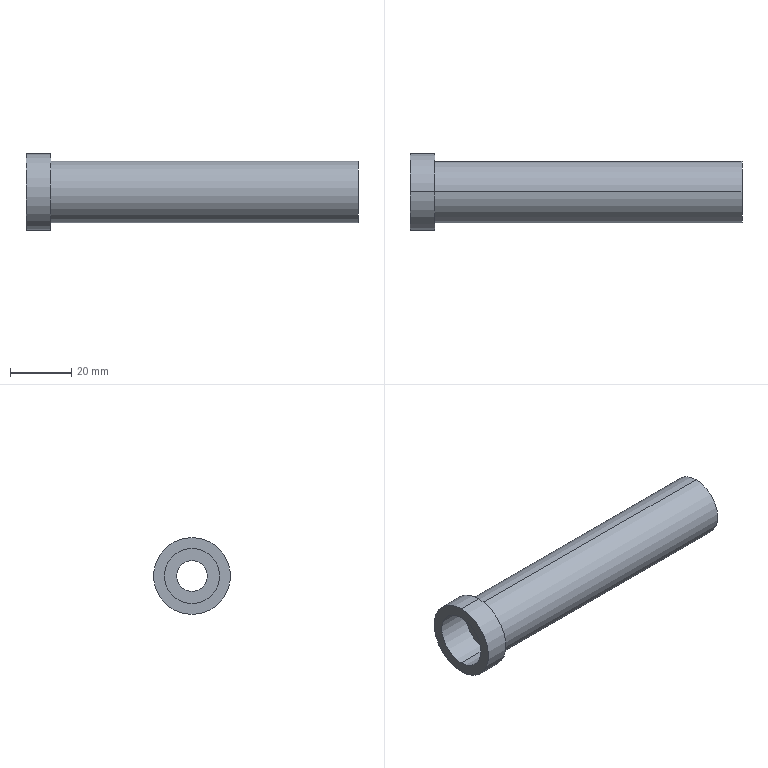Component | SolidWorks | ST60-13-1 | 1 solid | 12 faces | box 108 x 25 x 25 mm | volume 24925 mm3 | cylinder 8 | plane 4 | commonest cylinder face diameters 18 x2 10 x2 25 x2 20 x2
build123d program:
from build123d import *

# Parameters (mm, degrees)
SKETCH1_R                                          = 10
BOSS_EXTRUDE1_DEPTH                                = 100
SKETCH2_R                                          = 12.5
BOSS_EXTRUDE2_DEPTH                                = 8
HOLE_SIZE_ACCORDING_TO_TYPE_1_OF_HEXAG_D           = 10
HOLE_SIZE_ACCORDING_TO_TYPE_1_OF_HEXAG_CBORE_D     = 18
HOLE_SIZE_ACCORDING_TO_TYPE_1_OF_HEXAG_CBORE_DEPTH = 11


with BuildPart() as part:
    # Sketch1 → Boss-Extrude1 (new body)
    with BuildSketch(Plane.XY):
        Circle(SKETCH1_R)
    extrude(amount=BOSS_EXTRUDE1_DEPTH)

    # Sketch2 → Boss-Extrude2 (add)
    with BuildSketch(Plane.XY.offset(100)):
        Circle(SKETCH2_R)
    extrude(amount=BOSS_EXTRUDE2_DEPTH)

    # Hole Size _According to_ Type 1 of Hexag (through all)
    with Locations(Plane.XY.offset(108)):
        with Locations((0, 0)):
            CounterBoreHole(HOLE_SIZE_ACCORDING_TO_TYPE_1_OF_HEXAG_D / 2, HOLE_SIZE_ACCORDING_TO_TYPE_1_OF_HEXAG_CBORE_D / 2, HOLE_SIZE_ACCORDING_TO_TYPE_1_OF_HEXAG_CBORE_DEPTH)


solid = part.part

# Placed as in the assembly
solid = solid.moved(Location((259.993, 610.454, -1901.4), (0, -90, 0)))
STEP:
#1=COLOUR_RGB('',0.7922,0.8196,0.9333);
#2=FILL_AREA_STYLE_COLOUR('',#1);
#3=FILL_AREA_STYLE('',(#2));
#4=SURFACE_STYLE_FILL_AREA(#3);
#5=SURFACE_SIDE_STYLE('',(#4));
#6=SURFACE_STYLE_USAGE(.BOTH.,#5);
#7=PRESENTATION_STYLE_ASSIGNMENT((#6));
#8=CARTESIAN_POINT('',(6.417,24.034,-75.213));
#9=VERTEX_POINT('',#8);
#10=CARTESIAN_POINT('',(6.417,24.034,-74.504));
#11=VERTEX_POINT('',#10);
#12=CARTESIAN_POINT('',(6.417,24.034,-74.858));
#13=DIRECTION('',(-1.,-0.,0.));
#14=DIRECTION('',(0.,0.,1.));
#15=AXIS2_PLACEMENT_3D('',#12,#13,#14);
#16=CIRCLE('',#15,0.3543);
#17=EDGE_CURVE('',#9,#11,#16,.T.);
#18=ORIENTED_EDGE('',*,*,#17,.F.);
#19=CARTESIAN_POINT('',(5.984,24.034,-75.213));
#20=VERTEX_POINT('',#19);
#21=CARTESIAN_POINT('',(5.984,24.034,-75.213));
#22=DIRECTION('',(-1.,-0.,0.));
#23=VECTOR('',#22,39.37);
#24=LINE('',#21,#23);
#25=EDGE_CURVE('',#9,#20,#24,.T.);
#26=ORIENTED_EDGE('',*,*,#25,.T.);
#27=CARTESIAN_POINT('',(5.984,24.034,-74.504));
#28=VERTEX_POINT('',#27);
#29=CARTESIAN_POINT('',(5.984,24.034,-74.858));
#30=DIRECTION('',(-1.,-0.,0.));
#31=DIRECTION('',(0.,0.,1.));
#32=AXIS2_PLACEMENT_3D('',#29,#30,#31);
#33=CIRCLE('',#32,0.3543);
#34=EDGE_CURVE('',#20,#28,#33,.T.);
#35=ORIENTED_EDGE('',*,*,#34,.T.);
#36=CARTESIAN_POINT('',(5.984,24.034,-74.504));
#37=DIRECTION('',(-1.,-0.,0.));
#38=VECTOR('',#37,39.37);
#39=LINE('',#36,#38);
#40=EDGE_CURVE('',#11,#28,#39,.T.);
#41=ORIENTED_EDGE('',*,*,#40,.F.);
#42=EDGE_LOOP('',(#18,#26,#35,#41));
#43=FACE_OUTER_BOUND('',#42,.T.);
#44=CARTESIAN_POINT('',(5.984,24.034,-74.858));
#45=DIRECTION('',(-1.,-0.,0.));
#46=DIRECTION('',(0.,0.,1.));
#47=AXIS2_PLACEMENT_3D('',#44,#45,#46);
#48=CYLINDRICAL_SURFACE('',#47,0.3543);
#49=ADVANCED_FACE('',(#43),#48,.F.);
#50=CARTESIAN_POINT('',(10.236,24.034,-75.055));
#51=VERTEX_POINT('',#50);
#52=CARTESIAN_POINT('',(10.236,24.034,-74.661));
#53=VERTEX_POINT('',#52);
#54=CARTESIAN_POINT('',(10.236,24.034,-74.858));
#55=DIRECTION('',(-1.,-0.,0.));
#56=DIRECTION('',(0.,0.,1.));
#57=AXIS2_PLACEMENT_3D('',#54,#55,#56);
#58=CIRCLE('',#57,0.1969);
#59=EDGE_CURVE('',#51,#53,#58,.T.);
#60=ORIENTED_EDGE('',*,*,#59,.F.);
#61=CARTESIAN_POINT('',(6.417,24.034,-75.055));
#62=VERTEX_POINT('',#61);
#63=CARTESIAN_POINT('',(5.984,24.034,-75.055));
#64=DIRECTION('',(-1.,-0.,0.));
#65=VECTOR('',#64,39.37);
#66=LINE('',#63,#65);
#67=EDGE_CURVE('',#51,#62,#66,.T.);
#68=ORIENTED_EDGE('',*,*,#67,.T.);
#69=CARTESIAN_POINT('',(6.417,24.034,-74.661));
#70=VERTEX_POINT('',#69);
#71=CARTESIAN_POINT('',(6.417,24.034,-74.858));
#72=DIRECTION('',(-1.,-0.,0.));
#73=DIRECTION('',(0.,0.,1.));
#74=AXIS2_PLACEMENT_3D('',#71,#72,#73);
#75=CIRCLE('',#74,0.1969);
#76=EDGE_CURVE('',#62,#70,#75,.T.);
#77=ORIENTED_EDGE('',*,*,#76,.T.);
#78=CARTESIAN_POINT('',(5.984,24.034,-74.661));
#79=DIRECTION('',(-1.,-0.,0.));
#80=VECTOR('',#79,39.37);
#81=LINE('',#78,#80);
#82=EDGE_CURVE('',#53,#70,#81,.T.);
#83=ORIENTED_EDGE('',*,*,#82,.F.);
#84=EDGE_LOOP('',(#60,#68,#77,#83));
#85=FACE_OUTER_BOUND('',#84,.T.);
#86=CARTESIAN_POINT('',(5.984,24.034,-74.858));
#87=DIRECTION('',(-1.,-0.,0.));
#88=DIRECTION('',(0.,0.,1.));
#89=AXIS2_PLACEMENT_3D('',#86,#87,#88);
#90=CYLINDRICAL_SURFACE('',#89,0.1969);
#91=ADVANCED_FACE('',(#85),#90,.F.);
#92=CARTESIAN_POINT('',(5.984,24.034,-74.366));
#93=VERTEX_POINT('',#92);
#94=CARTESIAN_POINT('',(5.984,24.034,-75.35));
#95=VERTEX_POINT('',#94);
#96=CARTESIAN_POINT('',(5.984,24.034,-74.858));
#97=DIRECTION('',(-1.,-0.,0.));
#98=DIRECTION('',(0.,0.,1.));
#99=AXIS2_PLACEMENT_3D('',#96,#97,#98);
#100=CIRCLE('',#99,0.4921);
#101=EDGE_CURVE('',#93,#95,#100,.T.);
#102=ORIENTED_EDGE('',*,*,#101,.F.);
#103=CARTESIAN_POINT('',(6.299,24.034,-74.366));
#104=VERTEX_POINT('',#103);
#105=CARTESIAN_POINT('',(5.984,24.034,-74.366));
#106=DIRECTION('',(1.,0.,-0.));
#107=VECTOR('',#106,39.37);
#108=LINE('',#105,#107);
#109=EDGE_CURVE('',#93,#104,#108,.T.);
#110=ORIENTED_EDGE('',*,*,#109,.T.);
#111=CARTESIAN_POINT('',(6.299,24.034,-75.35));
#112=VERTEX_POINT('',#111);
#113=CARTESIAN_POINT('',(6.299,24.034,-74.858));
#114=DIRECTION('',(-1.,-0.,0.));
#115=DIRECTION('',(0.,0.,1.));
#116=AXIS2_PLACEMENT_3D('',#113,#114,#115);
#117=CIRCLE('',#116,0.4921);
#118=EDGE_CURVE('',#104,#112,#117,.T.);
#119=ORIENTED_EDGE('',*,*,#118,.T.);
#120=CARTESIAN_POINT('',(5.984,24.034,-75.35));
#121=DIRECTION('',(1.,0.,-0.));
#122=VECTOR('',#121,39.37);
#123=LINE('',#120,#122);
#124=EDGE_CURVE('',#95,#112,#123,.T.);
#125=ORIENTED_EDGE('',*,*,#124,.F.);
#126=EDGE_LOOP('',(#102,#110,#119,#125));
#127=FACE_OUTER_BOUND('',#126,.T.);
#128=CARTESIAN_POINT('',(5.984,24.034,-74.858));
#129=DIRECTION('',(1.,0.,-0.));
#130=DIRECTION('',(0.,0.,-1.));
#131=AXIS2_PLACEMENT_3D('',#128,#129,#130);
#132=CYLINDRICAL_SURFACE('',#131,0.4921);
#133=ADVANCED_FACE('',(#127),#132,.T.);
#134=CARTESIAN_POINT('',(6.299,24.034,-74.465));
#135=VERTEX_POINT('',#134);
#136=CARTESIAN_POINT('',(6.299,24.034,-75.252));
#137=VERTEX_POINT('',#136);
#138=CARTESIAN_POINT('',(6.299,24.034,-74.858));
#139=DIRECTION('',(-1.,-0.,0.));
#140=DIRECTION('',(0.,0.,1.));
#141=AXIS2_PLACEMENT_3D('',#138,#139,#140);
#142=CIRCLE('',#141,0.3937);
#143=EDGE_CURVE('',#135,#137,#142,.T.);
#144=ORIENTED_EDGE('',*,*,#143,.F.);
#145=CARTESIAN_POINT('',(10.236,24.034,-74.465));
#146=VERTEX_POINT('',#145);
#147=CARTESIAN_POINT('',(6.299,24.034,-74.465));
#148=DIRECTION('',(1.,0.,-0.));
#149=VECTOR('',#148,39.37);
#150=LINE('',#147,#149);
#151=EDGE_CURVE('',#135,#146,#150,.T.);
#152=ORIENTED_EDGE('',*,*,#151,.T.);
#153=CARTESIAN_POINT('',(10.236,24.034,-75.252));
#154=VERTEX_POINT('',#153);
#155=CARTESIAN_POINT('',(10.236,24.034,-74.858));
#156=DIRECTION('',(-1.,-0.,0.));
#157=DIRECTION('',(0.,0.,1.));
#158=AXIS2_PLACEMENT_3D('',#155,#156,#157);
#159=CIRCLE('',#158,0.3937);
#160=EDGE_CURVE('',#146,#154,#159,.T.);
#161=ORIENTED_EDGE('',*,*,#160,.T.);
#162=CARTESIAN_POINT('',(6.299,24.034,-75.252));
#163=DIRECTION('',(1.,0.,-0.));
#164=VECTOR('',#163,39.37);
#165=LINE('',#162,#164);
#166=EDGE_CURVE('',#137,#154,#165,.T.);
#167=ORIENTED_EDGE('',*,*,#166,.F.);
#168=EDGE_LOOP('',(#144,#152,#161,#167));
#169=FACE_OUTER_BOUND('',#168,.T.);
#170=CARTESIAN_POINT('',(6.299,24.034,-74.858));
#171=DIRECTION('',(1.,0.,-0.));
#172=DIRECTION('',(0.,0.,-1.));
#173=AXIS2_PLACEMENT_3D('',#170,#171,#172);
#174=CYLINDRICAL_SURFACE('',#173,0.3937);
#175=ADVANCED_FACE('',(#169),#174,.T.);
#176=ORIENTED_EDGE('',*,*,#151,.F.);
#177=CARTESIAN_POINT('',(6.299,24.034,-74.858));
#178=DIRECTION('',(-1.,-0.,0.));
#179=DIRECTION('',(0.,0.,1.));
#180=AXIS2_PLACEMENT_3D('',#177,#178,#179);
#181=CIRCLE('',#180,0.3937);
#182=EDGE_CURVE('',#137,#135,#181,.T.);
#183=ORIENTED_EDGE('',*,*,#182,.F.);
#184=ORIENTED_EDGE('',*,*,#166,.T.);
#185=CARTESIAN_POINT('',(10.236,24.034,-74.858));
#186=DIRECTION('',(-1.,-0.,0.));
#187=DIRECTION('',(0.,0.,1.));
#188=AXIS2_PLACEMENT_3D('',#185,#186,#187);
#189=CIRCLE('',#188,0.3937);
#190=EDGE_CURVE('',#154,#146,#189,.T.);
#191=ORIENTED_EDGE('',*,*,#190,.T.);
#192=EDGE_LOOP('',(#176,#183,#184,#191));
#193=FACE_OUTER_BOUND('',#192,.T.);
#194=CARTESIAN_POINT('',(6.299,24.034,-74.858));
#195=DIRECTION('',(1.,0.,-0.));
#196=DIRECTION('',(0.,0.,-1.));
#197=AXIS2_PLACEMENT_3D('',#194,#195,#196);
#198=CYLINDRICAL_SURFACE('',#197,0.3937);
#199=ADVANCED_FACE('',(#193),#198,.T.);
#200=CARTESIAN_POINT('',(10.236,24.034,-74.858));
#201=DIRECTION('',(-1.,-0.,0.));
#202=DIRECTION('',(0.,0.,1.));
#203=AXIS2_PLACEMENT_3D('',#200,#201,#202);
#204=CIRCLE('',#203,0.1969);
#205=EDGE_CURVE('',#53,#51,#204,.T.);
#206=ORIENTED_EDGE('',*,*,#205,.T.);
#207=ORIENTED_EDGE('',*,*,#59,.T.);
#208=EDGE_LOOP('',(#206,#207));
#209=FACE_BOUND('',#208,.T.);
#210=ORIENTED_EDGE('',*,*,#190,.F.);
#211=ORIENTED_EDGE('',*,*,#160,.F.);
#212=EDGE_LOOP('',(#210,#211));
#213=FACE_OUTER_BOUND('',#212,.T.);
#214=CARTESIAN_POINT('',(10.236,24.034,-74.858));
#215=DIRECTION('',(-1.,-0.,0.));
#216=DIRECTION('',(0.,0.,1.));
#217=AXIS2_PLACEMENT_3D('',#214,#215,#216);
#218=PLANE('',#217);
#219=ADVANCED_FACE('',(#209,#213),#218,.F.);
#220=ORIENTED_EDGE('',*,*,#109,.F.);
#221=CARTESIAN_POINT('',(5.984,24.034,-74.858));
#222=DIRECTION('',(-1.,-0.,0.));
#223=DIRECTION('',(0.,0.,1.));
#224=AXIS2_PLACEMENT_3D('',#221,#222,#223);
#225=CIRCLE('',#224,0.4921);
#226=EDGE_CURVE('',#95,#93,#225,.T.);
#227=ORIENTED_EDGE('',*,*,#226,.F.);
#228=ORIENTED_EDGE('',*,*,#124,.T.);
#229=CARTESIAN_POINT('',(6.299,24.034,-74.858));
#230=DIRECTION('',(-1.,-0.,0.));
#231=DIRECTION('',(0.,0.,1.));
#232=AXIS2_PLACEMENT_3D('',#229,#230,#231);
#233=CIRCLE('',#232,0.4921);
#234=EDGE_CURVE('',#112,#104,#233,.T.);
#235=ORIENTED_EDGE('',*,*,#234,.T.);
#236=EDGE_LOOP('',(#220,#227,#228,#235));
#237=FACE_OUTER_BOUND('',#236,.T.);
#238=CARTESIAN_POINT('',(5.984,24.034,-74.858));
#239=DIRECTION('',(1.,0.,-0.));
#240=DIRECTION('',(0.,0.,-1.));
#241=AXIS2_PLACEMENT_3D('',#238,#239,#240);
#242=CYLINDRICAL_SURFACE('',#241,0.4921);
#243=ADVANCED_FACE('',(#237),#242,.T.);
#244=CARTESIAN_POINT('',(5.984,24.034,-74.858));
#245=DIRECTION('',(-1.,-0.,0.));
#246=DIRECTION('',(0.,0.,1.));
#247=AXIS2_PLACEMENT_3D('',#244,#245,#246);
#248=CIRCLE('',#247,0.3543);
#249=EDGE_CURVE('',#28,#20,#248,.T.);
#250=ORIENTED_EDGE('',*,*,#249,.F.);
#251=ORIENTED_EDGE('',*,*,#34,.F.);
#252=EDGE_LOOP('',(#250,#251));
#253=FACE_BOUND('',#252,.T.);
#254=ORIENTED_EDGE('',*,*,#226,.T.);
#255=ORIENTED_EDGE('',*,*,#101,.T.);
#256=EDGE_LOOP('',(#254,#255));
#257=FACE_OUTER_BOUND('',#256,.T.);
#258=CARTESIAN_POINT('',(5.984,24.034,-74.858));
#259=DIRECTION('',(-1.,-0.,0.));
#260=DIRECTION('',(0.,0.,1.));
#261=AXIS2_PLACEMENT_3D('',#258,#259,#260);
#262=PLANE('',#261);
#263=ADVANCED_FACE('',(#253,#257),#262,.T.);
#264=ORIENTED_EDGE('',*,*,#182,.T.);
#265=ORIENTED_EDGE('',*,*,#143,.T.);
#266=EDGE_LOOP('',(#264,#265));
#267=FACE_BOUND('',#266,.T.);
#268=ORIENTED_EDGE('',*,*,#234,.F.);
#269=ORIENTED_EDGE('',*,*,#118,.F.);
#270=EDGE_LOOP('',(#268,#269));
#271=FACE_OUTER_BOUND('',#270,.T.);
#272=CARTESIAN_POINT('',(6.299,24.034,-74.858));
#273=DIRECTION('',(-1.,-0.,0.));
#274=DIRECTION('',(0.,0.,1.));
#275=AXIS2_PLACEMENT_3D('',#272,#273,#274);
#276=PLANE('',#275);
#277=ADVANCED_FACE('',(#267,#271),#276,.F.);
#278=ORIENTED_EDGE('',*,*,#67,.F.);
#279=ORIENTED_EDGE('',*,*,#205,.F.);
#280=ORIENTED_EDGE('',*,*,#82,.T.);
#281=CARTESIAN_POINT('',(6.417,24.034,-74.858));
#282=DIRECTION('',(-1.,-0.,0.));
#283=DIRECTION('',(0.,0.,1.));
#284=AXIS2_PLACEMENT_3D('',#281,#282,#283);
#285=CIRCLE('',#284,0.1969);
#286=EDGE_CURVE('',#70,#62,#285,.T.);
#287=ORIENTED_EDGE('',*,*,#286,.T.);
#288=EDGE_LOOP('',(#278,#279,#280,#287));
#289=FACE_OUTER_BOUND('',#288,.T.);
#290=CARTESIAN_POINT('',(5.984,24.034,-74.858));
#291=DIRECTION('',(-1.,-0.,0.));
#292=DIRECTION('',(0.,0.,1.));
#293=AXIS2_PLACEMENT_3D('',#290,#291,#292);
#294=CYLINDRICAL_SURFACE('',#293,0.1969);
#295=ADVANCED_FACE('',(#289),#294,.F.);
#296=ORIENTED_EDGE('',*,*,#286,.F.);
#297=ORIENTED_EDGE('',*,*,#76,.F.);
#298=EDGE_LOOP('',(#296,#297));
#299=FACE_BOUND('',#298,.T.);
#300=CARTESIAN_POINT('',(6.417,24.034,-74.858));
#301=DIRECTION('',(-1.,-0.,0.));
#302=DIRECTION('',(0.,0.,1.));
#303=AXIS2_PLACEMENT_3D('',#300,#301,#302);
#304=CIRCLE('',#303,0.3543);
#305=EDGE_CURVE('',#11,#9,#304,.T.);
#306=ORIENTED_EDGE('',*,*,#305,.T.);
#307=ORIENTED_EDGE('',*,*,#17,.T.);
#308=EDGE_LOOP('',(#306,#307));
#309=FACE_OUTER_BOUND('',#308,.T.);
#310=CARTESIAN_POINT('',(6.417,24.034,-74.661));
#311=DIRECTION('',(1.,0.,-0.));
#312=DIRECTION('',(-0.,-0.,-1.));
#313=AXIS2_PLACEMENT_3D('',#310,#311,#312);
#314=PLANE('',#313);
#315=ADVANCED_FACE('',(#299,#309),#314,.F.);
#316=ORIENTED_EDGE('',*,*,#25,.F.);
#317=ORIENTED_EDGE('',*,*,#305,.F.);
#318=ORIENTED_EDGE('',*,*,#40,.T.);
#319=ORIENTED_EDGE('',*,*,#249,.T.);
#320=EDGE_LOOP('',(#316,#317,#318,#319));
#321=FACE_OUTER_BOUND('',#320,.T.);
#322=CARTESIAN_POINT('',(5.984,24.034,-74.858));
#323=DIRECTION('',(-1.,-0.,0.));
#324=DIRECTION('',(0.,0.,1.));
#325=AXIS2_PLACEMENT_3D('',#322,#323,#324);
#326=CYLINDRICAL_SURFACE('',#325,0.3543);
#327=ADVANCED_FACE('',(#321),#326,.F.);
#328=CLOSED_SHELL('',(#49,#91,#133,#175,#199,#219,#243,#263,#277,#295,#315,#327));
#329=MANIFOLD_SOLID_BREP('',#328);
#330=STYLED_ITEM('',(#7),#329);
#331=(LENGTH_UNIT()NAMED_UNIT(*)SI_UNIT($,.METRE.));
#332=LENGTH_MEASURE_WITH_UNIT(LENGTH_MEASURE(0.0254),#331);
#333=DIMENSIONAL_EXPONENTS(1.,0.,0.,0.,0.,0.,0.);
#334=(CONVERSION_BASED_UNIT('',#332)LENGTH_UNIT()NAMED_UNIT(#333));
#335=UNCERTAINTY_MEASURE_WITH_UNIT(LENGTH_MEASURE(0.00001),#334,'','');
#336=(NAMED_UNIT(*)PLANE_ANGLE_UNIT()SI_UNIT($,.RADIAN.));
#337=(NAMED_UNIT(*)SI_UNIT($,.STERADIAN.)SOLID_ANGLE_UNIT());
#338=(GEOMETRIC_REPRESENTATION_CONTEXT(3)GLOBAL_UNCERTAINTY_ASSIGNED_CONTEXT((#335))GLOBAL_UNIT_ASSIGNED_CONTEXT((#334,#336,#337))REPRESENTATION_CONTEXT('',''));
#339=MECHANICAL_DESIGN_GEOMETRIC_PRESENTATION_REPRESENTATION('',(#330),#338);
#340=CARTESIAN_POINT('',(0.,0.,0.));
#341=DIRECTION('',(0.,0.,1.));
#342=DIRECTION('',(1.,0.,0.));
#343=AXIS2_PLACEMENT_3D('',#340,#341,#342);
#344=(LENGTH_UNIT()NAMED_UNIT(*)SI_UNIT($,.METRE.));
#345=LENGTH_MEASURE_WITH_UNIT(LENGTH_MEASURE(0.0254),#344);
#346=DIMENSIONAL_EXPONENTS(1.,0.,0.,0.,0.,0.,0.);
#347=(CONVERSION_BASED_UNIT('',#345)LENGTH_UNIT()NAMED_UNIT(#346));
#348=UNCERTAINTY_MEASURE_WITH_UNIT(LENGTH_MEASURE(0.00001),#347,'','');
#349=(NAMED_UNIT(*)PLANE_ANGLE_UNIT()SI_UNIT($,.RADIAN.));
#350=(NAMED_UNIT(*)SI_UNIT($,.STERADIAN.)SOLID_ANGLE_UNIT());
#351=(GEOMETRIC_REPRESENTATION_CONTEXT(3)GLOBAL_UNCERTAINTY_ASSIGNED_CONTEXT((#348))GLOBAL_UNIT_ASSIGNED_CONTEXT((#347,#349,#350))REPRESENTATION_CONTEXT('',''));
#352=ADVANCED_BREP_SHAPE_REPRESENTATION('',(#329,#343),#351);
#353=PRESENTATION_LAYER_ASSIGNMENT('','',(#330));